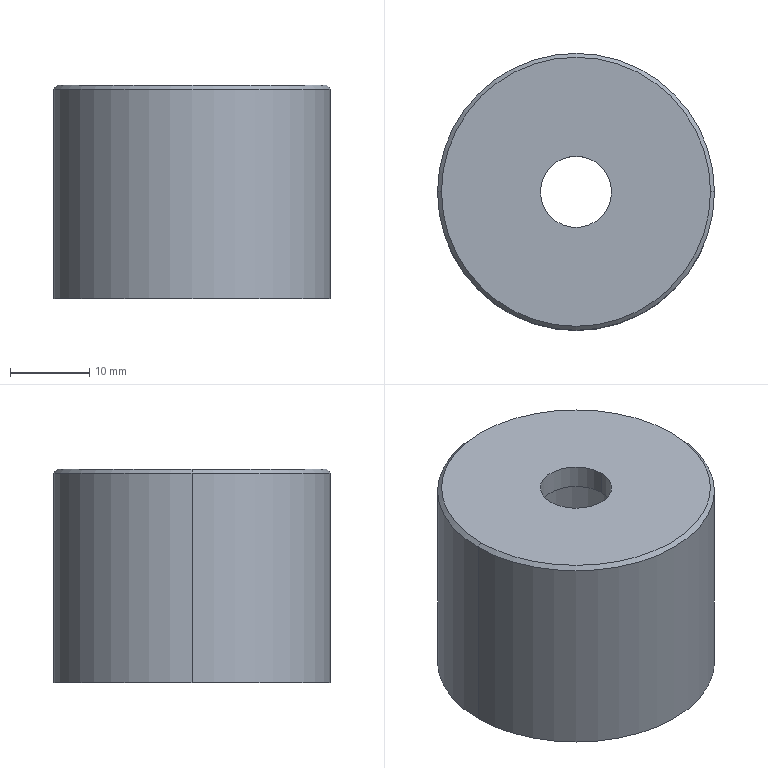Component | SolidWorks | YC1-250-03-01SliderAssembly-1_YC1-200-03-39SmallSprocketGland-1 | 1 solid | 14 faces | box 35 x 35 x 27 mm | volume 18292 mm3 | cylinder 6 | plane 4 | spline 2 | cone 2 | commonest cylinder face diameters 20 x2 35 x2 9 x2 | material Plain Carbon Steel
STEP:
#1=CARTESIAN_POINT('',(7.382,68.996,-11.339));
#2=VERTEX_POINT('',#1);
#3=CARTESIAN_POINT('',(6.791,68.996,-11.339));
#4=VERTEX_POINT('',#3);
#5=CARTESIAN_POINT('',(7.382,68.996,-11.339));
#6=CARTESIAN_POINT('',(7.382,69.587,-11.339));
#7=CARTESIAN_POINT('',(6.791,69.587,-11.339));
#8=CARTESIAN_POINT('',(6.791,68.996,-11.339));
#9=(BOUNDED_CURVE()B_SPLINE_CURVE(3,(#5,#6,#7,#8),.UNSPECIFIED.,.F.,.T.)B_SPLINE_CURVE_WITH_KNOTS((4,4),(0.,1.),.UNSPECIFIED.)CURVE()GEOMETRIC_REPRESENTATION_ITEM()RATIONAL_B_SPLINE_CURVE((1.,0.3333,0.3333,1.))REPRESENTATION_ITEM(''));
#10=EDGE_CURVE('',#2,#4,#9,.T.);
#11=ORIENTED_EDGE('',*,*,#10,.T.);
#12=CARTESIAN_POINT('',(6.772,68.996,-11.358));
#13=VERTEX_POINT('',#12);
#14=CARTESIAN_POINT('',(6.791,68.996,-11.358));
#15=DIRECTION('',(-0.,-1.,0.));
#16=DIRECTION('',(-1.,0.,0.));
#17=AXIS2_PLACEMENT_3D('',#14,#15,#16);
#18=CIRCLE('',#17,0.01969);
#19=EDGE_CURVE('',#4,#13,#18,.T.);
#20=ORIENTED_EDGE('',*,*,#19,.T.);
#21=CARTESIAN_POINT('',(7.402,68.996,-11.358));
#22=VERTEX_POINT('',#21);
#23=CARTESIAN_POINT('',(7.087,68.996,-11.358));
#24=DIRECTION('',(0.,0.,1.));
#25=DIRECTION('',(-1.,0.,0.));
#26=AXIS2_PLACEMENT_3D('',#23,#24,#25);
#27=CIRCLE('',#26,0.315);
#28=EDGE_CURVE('',#22,#13,#27,.T.);
#29=ORIENTED_EDGE('',*,*,#28,.F.);
#30=CARTESIAN_POINT('',(7.382,68.996,-11.358));
#31=DIRECTION('',(0.,1.,0.));
#32=DIRECTION('',(1.,0.,0.));
#33=AXIS2_PLACEMENT_3D('',#30,#31,#32);
#34=CIRCLE('',#33,0.01969);
#35=EDGE_CURVE('',#2,#22,#34,.T.);
#36=ORIENTED_EDGE('',*,*,#35,.F.);
#37=EDGE_LOOP('',(#11,#20,#29,#36));
#38=FACE_OUTER_BOUND('',#37,.T.);
#39=CARTESIAN_POINT('',(7.382,68.996,-11.339));
#40=CARTESIAN_POINT('',(7.382,69.587,-11.339));
#41=CARTESIAN_POINT('',(6.791,69.587,-11.339));
#42=CARTESIAN_POINT('',(6.791,68.996,-11.339));
#43=CARTESIAN_POINT('',(7.393,68.996,-11.339));
#44=CARTESIAN_POINT('',(7.393,69.61,-11.339));
#45=CARTESIAN_POINT('',(6.78,69.61,-11.339));
#46=CARTESIAN_POINT('',(6.78,68.996,-11.339));
#47=CARTESIAN_POINT('',(7.402,68.996,-11.347));
#48=CARTESIAN_POINT('',(7.402,69.626,-11.347));
#49=CARTESIAN_POINT('',(6.772,69.626,-11.347));
#50=CARTESIAN_POINT('',(6.772,68.996,-11.347));
#51=CARTESIAN_POINT('',(7.402,68.996,-11.358));
#52=CARTESIAN_POINT('',(7.402,69.626,-11.358));
#53=CARTESIAN_POINT('',(6.772,69.626,-11.358));
#54=CARTESIAN_POINT('',(6.772,68.996,-11.358));
#55=(BOUNDED_SURFACE()B_SPLINE_SURFACE(3,3,((#39,#40,#41,#42),(#43,#44,#45,#46),(#47,#48,#49,#50),(#51,#52,#53,#54)),.UNSPECIFIED.,.F.,.F.,.F.)B_SPLINE_SURFACE_WITH_KNOTS((4,4),(4,4),(0.,1.),(0.,1.),.UNSPECIFIED.)GEOMETRIC_REPRESENTATION_ITEM()RATIONAL_B_SPLINE_SURFACE(((1.,0.3333,0.3333,1.),(0.8047,0.2682,0.2682,0.8047),(0.8047,0.2682,0.2682,0.8047),(1.,0.3333,0.3333,1.)))REPRESENTATION_ITEM('')SURFACE());
#56=ADVANCED_FACE('',(#38),#55,.F.);
#57=CARTESIAN_POINT('',(7.48,68.996,-11.358));
#58=VERTEX_POINT('',#57);
#59=CARTESIAN_POINT('',(6.693,68.996,-11.358));
#60=VERTEX_POINT('',#59);
#61=CARTESIAN_POINT('',(7.087,68.996,-11.358));
#62=DIRECTION('',(0.,0.,-1.));
#63=DIRECTION('',(-1.,0.,0.));
#64=AXIS2_PLACEMENT_3D('',#61,#62,#63);
#65=CIRCLE('',#64,0.3937);
#66=EDGE_CURVE('',#58,#60,#65,.T.);
#67=ORIENTED_EDGE('',*,*,#66,.F.);
#68=CARTESIAN_POINT('',(7.48,68.996,-12.283));
#69=VERTEX_POINT('',#68);
#70=CARTESIAN_POINT('',(7.48,68.996,-11.22));
#71=DIRECTION('',(0.,0.,-1.));
#72=VECTOR('',#71,39.37);
#73=LINE('',#70,#72);
#74=EDGE_CURVE('',#58,#69,#73,.T.);
#75=ORIENTED_EDGE('',*,*,#74,.T.);
#76=CARTESIAN_POINT('',(6.693,68.996,-12.283));
#77=VERTEX_POINT('',#76);
#78=CARTESIAN_POINT('',(7.087,68.996,-12.283));
#79=DIRECTION('',(0.,0.,-1.));
#80=DIRECTION('',(1.,0.,0.));
#81=AXIS2_PLACEMENT_3D('',#78,#79,#80);
#82=CIRCLE('',#81,0.3937);
#83=EDGE_CURVE('',#69,#77,#82,.T.);
#84=ORIENTED_EDGE('',*,*,#83,.T.);
#85=CARTESIAN_POINT('',(6.693,68.996,-11.22));
#86=DIRECTION('',(0.,0.,-1.));
#87=VECTOR('',#86,39.37);
#88=LINE('',#85,#87);
#89=EDGE_CURVE('',#60,#77,#88,.T.);
#90=ORIENTED_EDGE('',*,*,#89,.F.);
#91=EDGE_LOOP('',(#67,#75,#84,#90));
#92=FACE_OUTER_BOUND('',#91,.T.);
#93=CARTESIAN_POINT('',(7.087,68.996,-11.22));
#94=DIRECTION('',(0.,0.,-1.));
#95=DIRECTION('',(-1.,0.,0.));
#96=AXIS2_PLACEMENT_3D('',#93,#94,#95);
#97=CYLINDRICAL_SURFACE('',#96,0.3937);
#98=ADVANCED_FACE('',(#92),#97,.F.);
#99=CARTESIAN_POINT('',(7.776,68.996,-12.283));
#100=VERTEX_POINT('',#99);
#101=CARTESIAN_POINT('',(6.398,68.996,-12.283));
#102=VERTEX_POINT('',#101);
#103=CARTESIAN_POINT('',(7.087,68.996,-12.283));
#104=DIRECTION('',(0.,0.,1.));
#105=DIRECTION('',(1.,0.,0.));
#106=AXIS2_PLACEMENT_3D('',#103,#104,#105);
#107=CIRCLE('',#106,0.689);
#108=EDGE_CURVE('',#100,#102,#107,.T.);
#109=ORIENTED_EDGE('',*,*,#108,.T.);
#110=CARTESIAN_POINT('',(6.398,68.996,-11.24));
#111=VERTEX_POINT('',#110);
#112=CARTESIAN_POINT('',(6.398,68.996,-11.22));
#113=DIRECTION('',(0.,0.,1.));
#114=VECTOR('',#113,39.37);
#115=LINE('',#112,#114);
#116=EDGE_CURVE('',#102,#111,#115,.T.);
#117=ORIENTED_EDGE('',*,*,#116,.T.);
#118=CARTESIAN_POINT('',(7.776,68.996,-11.24));
#119=VERTEX_POINT('',#118);
#120=CARTESIAN_POINT('',(7.087,68.996,-11.24));
#121=DIRECTION('',(0.,0.,-1.));
#122=DIRECTION('',(1.,0.,0.));
#123=AXIS2_PLACEMENT_3D('',#120,#121,#122);
#124=CIRCLE('',#123,0.689);
#125=EDGE_CURVE('',#111,#119,#124,.T.);
#126=ORIENTED_EDGE('',*,*,#125,.T.);
#127=CARTESIAN_POINT('',(7.776,68.996,-11.22));
#128=DIRECTION('',(0.,0.,1.));
#129=VECTOR('',#128,39.37);
#130=LINE('',#127,#129);
#131=EDGE_CURVE('',#100,#119,#130,.T.);
#132=ORIENTED_EDGE('',*,*,#131,.F.);
#133=EDGE_LOOP('',(#109,#117,#126,#132));
#134=FACE_OUTER_BOUND('',#133,.T.);
#135=CARTESIAN_POINT('',(7.087,68.996,-11.22));
#136=DIRECTION('',(0.,0.,1.));
#137=DIRECTION('',(1.,0.,0.));
#138=AXIS2_PLACEMENT_3D('',#135,#136,#137);
#139=CYLINDRICAL_SURFACE('',#138,0.689);
#140=ADVANCED_FACE('',(#134),#139,.T.);
#141=CARTESIAN_POINT('',(6.417,68.996,-11.22));
#142=VERTEX_POINT('',#141);
#143=CARTESIAN_POINT('',(7.756,68.996,-11.22));
#144=VERTEX_POINT('',#143);
#145=CARTESIAN_POINT('',(7.087,68.996,-11.22));
#146=DIRECTION('',(0.,0.,-1.));
#147=DIRECTION('',(-1.,0.,0.));
#148=AXIS2_PLACEMENT_3D('',#145,#146,#147);
#149=CIRCLE('',#148,0.6693);
#150=EDGE_CURVE('',#142,#144,#149,.T.);
#151=ORIENTED_EDGE('',*,*,#150,.T.);
#152=CARTESIAN_POINT('',(7.776,68.996,-11.24));
#153=DIRECTION('',(0.7071,0.,-0.7071));
#154=VECTOR('',#153,39.37);
#155=LINE('',#152,#154);
#156=EDGE_CURVE('',#144,#119,#155,.T.);
#157=ORIENTED_EDGE('',*,*,#156,.T.);
#158=ORIENTED_EDGE('',*,*,#125,.F.);
#159=CARTESIAN_POINT('',(6.398,68.996,-11.24));
#160=DIRECTION('',(-0.7071,0.,-0.7071));
#161=VECTOR('',#160,39.37);
#162=LINE('',#159,#161);
#163=EDGE_CURVE('',#142,#111,#162,.T.);
#164=ORIENTED_EDGE('',*,*,#163,.F.);
#165=EDGE_LOOP('',(#151,#157,#158,#164));
#166=FACE_OUTER_BOUND('',#165,.T.);
#167=CARTESIAN_POINT('',(7.087,68.996,-11.24));
#168=DIRECTION('',(0.,0.,-1.));
#169=DIRECTION('',(-1.,0.,0.));
#170=AXIS2_PLACEMENT_3D('',#167,#168,#169);
#171=CONICAL_SURFACE('',#170,0.689,0.7854);
#172=ADVANCED_FACE('',(#166),#171,.T.);
#173=CARTESIAN_POINT('',(6.909,68.996,-11.339));
#174=VERTEX_POINT('',#173);
#175=CARTESIAN_POINT('',(7.264,68.996,-11.339));
#176=VERTEX_POINT('',#175);
#177=CARTESIAN_POINT('',(7.087,68.996,-11.339));
#178=DIRECTION('',(0.,0.,1.));
#179=DIRECTION('',(1.,0.,0.));
#180=AXIS2_PLACEMENT_3D('',#177,#178,#179);
#181=CIRCLE('',#180,0.1772);
#182=EDGE_CURVE('',#174,#176,#181,.T.);
#183=ORIENTED_EDGE('',*,*,#182,.F.);
#184=CARTESIAN_POINT('',(6.909,68.996,-11.22));
#185=VERTEX_POINT('',#184);
#186=CARTESIAN_POINT('',(6.909,68.996,-11.22));
#187=DIRECTION('',(0.,0.,1.));
#188=VECTOR('',#187,39.37);
#189=LINE('',#186,#188);
#190=EDGE_CURVE('',#174,#185,#189,.T.);
#191=ORIENTED_EDGE('',*,*,#190,.T.);
#192=CARTESIAN_POINT('',(7.264,68.996,-11.22));
#193=VERTEX_POINT('',#192);
#194=CARTESIAN_POINT('',(7.087,68.996,-11.22));
#195=DIRECTION('',(0.,0.,1.));
#196=DIRECTION('',(1.,0.,0.));
#197=AXIS2_PLACEMENT_3D('',#194,#195,#196);
#198=CIRCLE('',#197,0.1772);
#199=EDGE_CURVE('',#185,#193,#198,.T.);
#200=ORIENTED_EDGE('',*,*,#199,.T.);
#201=CARTESIAN_POINT('',(7.264,68.996,-11.22));
#202=DIRECTION('',(0.,0.,1.));
#203=VECTOR('',#202,39.37);
#204=LINE('',#201,#203);
#205=EDGE_CURVE('',#176,#193,#204,.T.);
#206=ORIENTED_EDGE('',*,*,#205,.F.);
#207=EDGE_LOOP('',(#183,#191,#200,#206));
#208=FACE_OUTER_BOUND('',#207,.T.);
#209=CARTESIAN_POINT('',(7.087,68.996,-11.22));
#210=DIRECTION('',(0.,0.,1.));
#211=DIRECTION('',(1.,0.,0.));
#212=AXIS2_PLACEMENT_3D('',#209,#210,#211);
#213=CYLINDRICAL_SURFACE('',#212,0.1772);
#214=ADVANCED_FACE('',(#208),#213,.F.);
#215=ORIENTED_EDGE('',*,*,#116,.F.);
#216=CARTESIAN_POINT('',(7.087,68.996,-12.283));
#217=DIRECTION('',(0.,0.,1.));
#218=DIRECTION('',(1.,0.,0.));
#219=AXIS2_PLACEMENT_3D('',#216,#217,#218);
#220=CIRCLE('',#219,0.689);
#221=EDGE_CURVE('',#102,#100,#220,.T.);
#222=ORIENTED_EDGE('',*,*,#221,.T.);
#223=ORIENTED_EDGE('',*,*,#131,.T.);
#224=CARTESIAN_POINT('',(7.087,68.996,-11.24));
#225=DIRECTION('',(0.,0.,-1.));
#226=DIRECTION('',(1.,0.,0.));
#227=AXIS2_PLACEMENT_3D('',#224,#225,#226);
#228=CIRCLE('',#227,0.689);
#229=EDGE_CURVE('',#119,#111,#228,.T.);
#230=ORIENTED_EDGE('',*,*,#229,.T.);
#231=EDGE_LOOP('',(#215,#222,#223,#230));
#232=FACE_OUTER_BOUND('',#231,.T.);
#233=CARTESIAN_POINT('',(7.087,68.996,-11.22));
#234=DIRECTION('',(0.,0.,1.));
#235=DIRECTION('',(1.,0.,0.));
#236=AXIS2_PLACEMENT_3D('',#233,#234,#235);
#237=CYLINDRICAL_SURFACE('',#236,0.689);
#238=ADVANCED_FACE('',(#232),#237,.T.);
#239=ORIENTED_EDGE('',*,*,#156,.F.);
#240=CARTESIAN_POINT('',(7.087,68.996,-11.22));
#241=DIRECTION('',(0.,0.,-1.));
#242=DIRECTION('',(-1.,0.,0.));
#243=AXIS2_PLACEMENT_3D('',#240,#241,#242);
#244=CIRCLE('',#243,0.6693);
#245=EDGE_CURVE('',#144,#142,#244,.T.);
#246=ORIENTED_EDGE('',*,*,#245,.T.);
#247=ORIENTED_EDGE('',*,*,#163,.T.);
#248=ORIENTED_EDGE('',*,*,#229,.F.);
#249=EDGE_LOOP('',(#239,#246,#247,#248));
#250=FACE_OUTER_BOUND('',#249,.T.);
#251=CARTESIAN_POINT('',(7.087,68.996,-11.24));
#252=DIRECTION('',(0.,0.,-1.));
#253=DIRECTION('',(-1.,0.,0.));
#254=AXIS2_PLACEMENT_3D('',#251,#252,#253);
#255=CONICAL_SURFACE('',#254,0.689,0.7854);
#256=ADVANCED_FACE('',(#250),#255,.T.);
#257=CARTESIAN_POINT('',(7.087,68.996,-12.283));
#258=DIRECTION('',(0.,0.,-1.));
#259=DIRECTION('',(1.,0.,0.));
#260=AXIS2_PLACEMENT_3D('',#257,#258,#259);
#261=CIRCLE('',#260,0.3937);
#262=EDGE_CURVE('',#77,#69,#261,.T.);
#263=ORIENTED_EDGE('',*,*,#262,.F.);
#264=ORIENTED_EDGE('',*,*,#83,.F.);
#265=EDGE_LOOP('',(#263,#264));
#266=FACE_BOUND('',#265,.T.);
#267=ORIENTED_EDGE('',*,*,#108,.F.);
#268=ORIENTED_EDGE('',*,*,#221,.F.);
#269=EDGE_LOOP('',(#267,#268));
#270=FACE_OUTER_BOUND('',#269,.T.);
#271=CARTESIAN_POINT('',(7.087,69.685,-12.283));
#272=DIRECTION('',(0.,0.,1.));
#273=DIRECTION('',(1.,0.,0.));
#274=AXIS2_PLACEMENT_3D('',#271,#272,#273);
#275=PLANE('',#274);
#276=ADVANCED_FACE('',(#266,#270),#275,.F.);
#277=ORIENTED_EDGE('',*,*,#150,.F.);
#278=ORIENTED_EDGE('',*,*,#245,.F.);
#279=EDGE_LOOP('',(#277,#278));
#280=FACE_OUTER_BOUND('',#279,.T.);
#281=CARTESIAN_POINT('',(7.087,68.996,-11.22));
#282=DIRECTION('',(0.,0.,1.));
#283=DIRECTION('',(1.,0.,0.));
#284=AXIS2_PLACEMENT_3D('',#281,#282,#283);
#285=CIRCLE('',#284,0.1772);
#286=EDGE_CURVE('',#193,#185,#285,.T.);
#287=ORIENTED_EDGE('',*,*,#286,.F.);
#288=ORIENTED_EDGE('',*,*,#199,.F.);
#289=EDGE_LOOP('',(#287,#288));
#290=FACE_BOUND('',#289,.T.);
#291=CARTESIAN_POINT('',(7.087,68.996,-11.22));
#292=DIRECTION('',(0.,0.,-1.));
#293=DIRECTION('',(-1.,0.,0.));
#294=AXIS2_PLACEMENT_3D('',#291,#292,#293);
#295=PLANE('',#294);
#296=ADVANCED_FACE('',(#280,#290),#295,.F.);
#297=ORIENTED_EDGE('',*,*,#190,.F.);
#298=CARTESIAN_POINT('',(7.087,68.996,-11.339));
#299=DIRECTION('',(0.,0.,1.));
#300=DIRECTION('',(1.,0.,0.));
#301=AXIS2_PLACEMENT_3D('',#298,#299,#300);
#302=CIRCLE('',#301,0.1772);
#303=EDGE_CURVE('',#176,#174,#302,.T.);
#304=ORIENTED_EDGE('',*,*,#303,.F.);
#305=ORIENTED_EDGE('',*,*,#205,.T.);
#306=ORIENTED_EDGE('',*,*,#286,.T.);
#307=EDGE_LOOP('',(#297,#304,#305,#306));
#308=FACE_OUTER_BOUND('',#307,.T.);
#309=CARTESIAN_POINT('',(7.087,68.996,-11.22));
#310=DIRECTION('',(0.,0.,1.));
#311=DIRECTION('',(1.,0.,0.));
#312=AXIS2_PLACEMENT_3D('',#309,#310,#311);
#313=CYLINDRICAL_SURFACE('',#312,0.1772);
#314=ADVANCED_FACE('',(#308),#313,.F.);
#315=ORIENTED_EDGE('',*,*,#10,.F.);
#316=CARTESIAN_POINT('',(6.791,68.996,-11.339));
#317=CARTESIAN_POINT('',(6.791,68.406,-11.339));
#318=CARTESIAN_POINT('',(7.382,68.406,-11.339));
#319=CARTESIAN_POINT('',(7.382,68.996,-11.339));
#320=(BOUNDED_CURVE()B_SPLINE_CURVE(3,(#316,#317,#318,#319),.UNSPECIFIED.,.F.,.T.)B_SPLINE_CURVE_WITH_KNOTS((4,4),(0.,1.),.UNSPECIFIED.)CURVE()GEOMETRIC_REPRESENTATION_ITEM()RATIONAL_B_SPLINE_CURVE((1.,0.3333,0.3333,1.))REPRESENTATION_ITEM(''));
#321=EDGE_CURVE('',#4,#2,#320,.T.);
#322=ORIENTED_EDGE('',*,*,#321,.F.);
#323=EDGE_LOOP('',(#315,#322));
#324=FACE_OUTER_BOUND('',#323,.T.);
#325=ORIENTED_EDGE('',*,*,#303,.T.);
#326=ORIENTED_EDGE('',*,*,#182,.T.);
#327=EDGE_LOOP('',(#325,#326));
#328=FACE_BOUND('',#327,.T.);
#329=CARTESIAN_POINT('',(7.087,69.311,-11.339));
#330=DIRECTION('',(0.,0.,1.));
#331=DIRECTION('',(1.,0.,0.));
#332=AXIS2_PLACEMENT_3D('',#329,#330,#331);
#333=PLANE('',#332);
#334=ADVANCED_FACE('',(#324,#328),#333,.F.);
#335=ORIENTED_EDGE('',*,*,#19,.F.);
#336=ORIENTED_EDGE('',*,*,#321,.T.);
#337=ORIENTED_EDGE('',*,*,#35,.T.);
#338=CARTESIAN_POINT('',(7.087,68.996,-11.358));
#339=DIRECTION('',(0.,0.,1.));
#340=DIRECTION('',(-1.,0.,0.));
#341=AXIS2_PLACEMENT_3D('',#338,#339,#340);
#342=CIRCLE('',#341,0.315);
#343=EDGE_CURVE('',#13,#22,#342,.T.);
#344=ORIENTED_EDGE('',*,*,#343,.F.);
#345=EDGE_LOOP('',(#335,#336,#337,#344));
#346=FACE_OUTER_BOUND('',#345,.T.);
#347=CARTESIAN_POINT('',(6.791,68.996,-11.339));
#348=CARTESIAN_POINT('',(6.791,68.406,-11.339));
#349=CARTESIAN_POINT('',(7.382,68.406,-11.339));
#350=CARTESIAN_POINT('',(7.382,68.996,-11.339));
#351=CARTESIAN_POINT('',(6.78,68.996,-11.339));
#352=CARTESIAN_POINT('',(6.78,68.382,-11.339));
#353=CARTESIAN_POINT('',(7.393,68.382,-11.339));
#354=CARTESIAN_POINT('',(7.393,68.996,-11.339));
#355=CARTESIAN_POINT('',(6.772,68.996,-11.347));
#356=CARTESIAN_POINT('',(6.772,68.366,-11.347));
#357=CARTESIAN_POINT('',(7.402,68.366,-11.347));
#358=CARTESIAN_POINT('',(7.402,68.996,-11.347));
#359=CARTESIAN_POINT('',(6.772,68.996,-11.358));
#360=CARTESIAN_POINT('',(6.772,68.366,-11.358));
#361=CARTESIAN_POINT('',(7.402,68.366,-11.358));
#362=CARTESIAN_POINT('',(7.402,68.996,-11.358));
#363=(BOUNDED_SURFACE()B_SPLINE_SURFACE(3,3,((#347,#348,#349,#350),(#351,#352,#353,#354),(#355,#356,#357,#358),(#359,#360,#361,#362)),.UNSPECIFIED.,.F.,.F.,.T.)B_SPLINE_SURFACE_WITH_KNOTS((4,4),(4,4),(0.,1.),(0.,1.),.UNSPECIFIED.)GEOMETRIC_REPRESENTATION_ITEM()RATIONAL_B_SPLINE_SURFACE(((1.,0.3333,0.3333,1.),(0.8047,0.2682,0.2682,0.8047),(0.8047,0.2682,0.2682,0.8047),(1.,0.3333,0.3333,1.)))REPRESENTATION_ITEM('')SURFACE());
#364=ADVANCED_FACE('',(#346),#363,.F.);
#365=CARTESIAN_POINT('',(7.087,68.996,-11.358));
#366=DIRECTION('',(0.,0.,-1.));
#367=DIRECTION('',(-1.,0.,0.));
#368=AXIS2_PLACEMENT_3D('',#365,#366,#367);
#369=CIRCLE('',#368,0.3937);
#370=EDGE_CURVE('',#60,#58,#369,.T.);
#371=ORIENTED_EDGE('',*,*,#370,.T.);
#372=ORIENTED_EDGE('',*,*,#66,.T.);
#373=EDGE_LOOP('',(#371,#372));
#374=FACE_OUTER_BOUND('',#373,.T.);
#375=ORIENTED_EDGE('',*,*,#28,.T.);
#376=ORIENTED_EDGE('',*,*,#343,.T.);
#377=EDGE_LOOP('',(#375,#376));
#378=FACE_BOUND('',#377,.T.);
#379=CARTESIAN_POINT('',(7.48,68.996,-11.358));
#380=DIRECTION('',(0.,0.,-1.));
#381=DIRECTION('',(-1.,0.,0.));
#382=AXIS2_PLACEMENT_3D('',#379,#380,#381);
#383=PLANE('',#382);
#384=ADVANCED_FACE('',(#374,#378),#383,.T.);
#385=ORIENTED_EDGE('',*,*,#74,.F.);
#386=ORIENTED_EDGE('',*,*,#370,.F.);
#387=ORIENTED_EDGE('',*,*,#89,.T.);
#388=ORIENTED_EDGE('',*,*,#262,.T.);
#389=EDGE_LOOP('',(#385,#386,#387,#388));
#390=FACE_OUTER_BOUND('',#389,.T.);
#391=CARTESIAN_POINT('',(7.087,68.996,-11.22));
#392=DIRECTION('',(0.,0.,-1.));
#393=DIRECTION('',(-1.,0.,0.));
#394=AXIS2_PLACEMENT_3D('',#391,#392,#393);
#395=CYLINDRICAL_SURFACE('',#394,0.3937);
#396=ADVANCED_FACE('',(#390),#395,.F.);
#397=CLOSED_SHELL('',(#56,#98,#140,#172,#214,#238,#256,#276,#296,#314,#334,#364,#384,#396));
#398=MANIFOLD_SOLID_BREP('',#397);
#399=CARTESIAN_POINT('',(0.,0.,0.));
#400=DIRECTION('',(0.,0.,1.));
#401=DIRECTION('',(1.,0.,0.));
#402=AXIS2_PLACEMENT_3D('',#399,#400,#401);
#403=(LENGTH_UNIT()NAMED_UNIT(*)SI_UNIT($,.METRE.));
#404=LENGTH_MEASURE_WITH_UNIT(LENGTH_MEASURE(0.0254),#403);
#405=DIMENSIONAL_EXPONENTS(1.,0.,0.,0.,0.,0.,0.);
#406=(CONVERSION_BASED_UNIT('',#404)LENGTH_UNIT()NAMED_UNIT(#405));
#407=UNCERTAINTY_MEASURE_WITH_UNIT(LENGTH_MEASURE(0.00001),#406,'','');
#408=(NAMED_UNIT(*)PLANE_ANGLE_UNIT()SI_UNIT($,.RADIAN.));
#409=(NAMED_UNIT(*)SI_UNIT($,.STERADIAN.)SOLID_ANGLE_UNIT());
#410=(GEOMETRIC_REPRESENTATION_CONTEXT(3)GLOBAL_UNCERTAINTY_ASSIGNED_CONTEXT((#407))GLOBAL_UNIT_ASSIGNED_CONTEXT((#406,#408,#409))REPRESENTATION_CONTEXT('',''));
#411=ADVANCED_BREP_SHAPE_REPRESENTATION('',(#398,#402),#410);
#412=COLOUR_RGB('',0.7922,0.8196,0.9333);
#413=FILL_AREA_STYLE_COLOUR('',#412);
#414=FILL_AREA_STYLE('',(#413));
#415=SURFACE_STYLE_FILL_AREA(#414);
#416=SURFACE_SIDE_STYLE('',(#415));
#417=SURFACE_STYLE_USAGE(.BOTH.,#416);
#418=PRESENTATION_STYLE_ASSIGNMENT((#417));
#419=STYLED_ITEM('',(#418),#398);
#420=PRESENTATION_LAYER_ASSIGNMENT('','',(#419));
#421=(LENGTH_UNIT()NAMED_UNIT(*)SI_UNIT($,.METRE.));
#422=LENGTH_MEASURE_WITH_UNIT(LENGTH_MEASURE(0.0254),#421);
#423=DIMENSIONAL_EXPONENTS(1.,0.,0.,0.,0.,0.,0.);
#424=(CONVERSION_BASED_UNIT('',#422)LENGTH_UNIT()NAMED_UNIT(#423));
#425=UNCERTAINTY_MEASURE_WITH_UNIT(LENGTH_MEASURE(0.00001),#424,'','');
#426=(NAMED_UNIT(*)PLANE_ANGLE_UNIT()SI_UNIT($,.RADIAN.));
#427=(NAMED_UNIT(*)SI_UNIT($,.STERADIAN.)SOLID_ANGLE_UNIT());
#428=(GEOMETRIC_REPRESENTATION_CONTEXT(3)GLOBAL_UNCERTAINTY_ASSIGNED_CONTEXT((#425))GLOBAL_UNIT_ASSIGNED_CONTEXT((#424,#426,#427))REPRESENTATION_CONTEXT('',''));
#429=MECHANICAL_DESIGN_GEOMETRIC_PRESENTATION_REPRESENTATION('',(#419),#428);